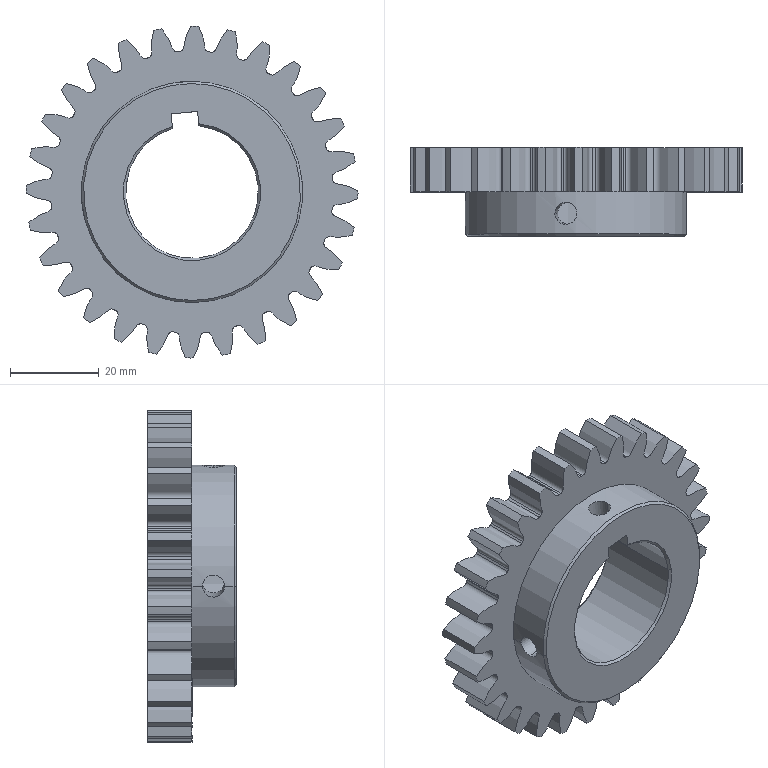Component | SolidWorks | 28zGear-1 | 1 solid | 136 faces | volume 42871 mm3 | cylinder 66 | spline 56 | cone 8 | plane 6 | commonest cylinder face diameters 63.75 x29 75 x28 5 x4 30 x3 50 x2